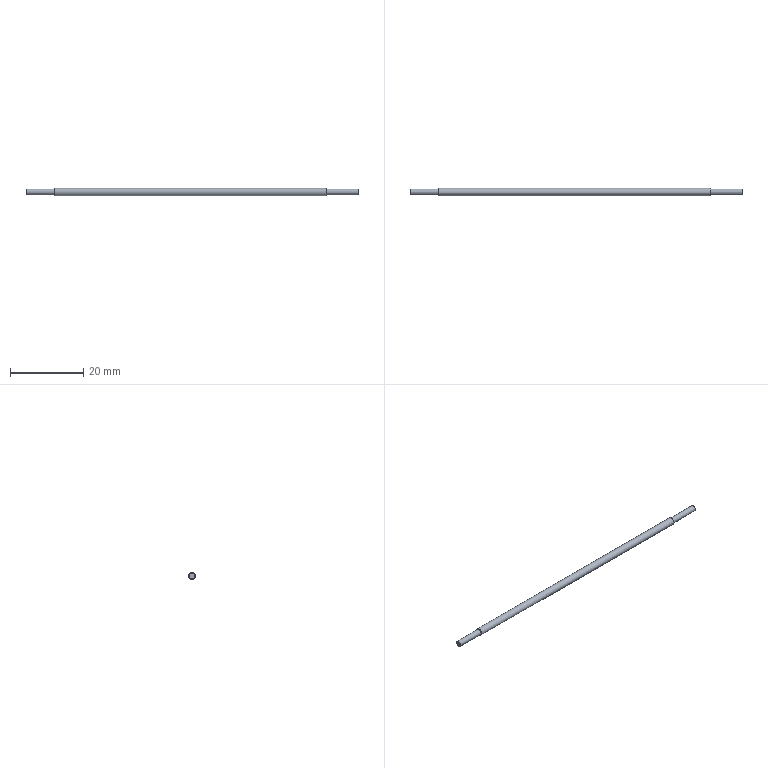Component | NX | LONG_SHAFT | 1 solid | 7 faces | box 90.9 x 2 x 2 mm | volume 267 mm3 | plane 4 | cylinder 3 | commonest cylinder face diameters 1.6 x2 2 x1
STEP:
#1=CARTESIAN_POINT('',(0.,0.,0.));
#2=DIRECTION('',(0.,0.,1.));
#3=DIRECTION('',(1.,0.,0.));
#4=AXIS2_PLACEMENT_3D('',#1,#2,#3);
#5=CARTESIAN_POINT('',(-47.4,2.21,6.167));
#6=VERTEX_POINT('',#5);
#7=CARTESIAN_POINT('',(-47.4,0.6405,6.477));
#8=VERTEX_POINT('',#7);
#9=CARTESIAN_POINT('',(-47.4,1.425,6.322));
#10=DIRECTION('',(-1.,0.,-0.));
#11=DIRECTION('',(0.,0.9811,-0.1935));
#12=AXIS2_PLACEMENT_3D('',#9,#10,#11);
#13=CIRCLE('',#12,0.8);
#14=CARTESIAN_POINT('',(-47.4,1.425,6.322));
#15=DIRECTION('',(1.,-0.,0.));
#16=DIRECTION('',(0.,0.00581,-1.));
#17=AXIS2_PLACEMENT_3D('',#14,#15,#16);
#18=PLANE('',#17);
#19=CARTESIAN_POINT('',(0.1594,0.784));
#20=CARTESIAN_POINT('',(1.517,0.508));
#21=CARTESIAN_POINT('',(0.5993,-0.53));
#22=CARTESIAN_POINT('',(-0.3187,-1.568));
#23=CARTESIAN_POINT('',(-0.7586,-0.254));
#24=CARTESIAN_POINT('',(-1.199,1.06));
#25=CARTESIAN_POINT('',(0.1594,0.784));
#26=(BOUNDED_CURVE()B_SPLINE_CURVE(2,(#19,#20,#21,#22,#23,#24,#25),.UNSPECIFIED.,.T.,.F.)B_SPLINE_CURVE_WITH_KNOTS((1,2,2,2,2,1),(-2.094,0.,2.094,4.189,6.283,8.378),.UNSPECIFIED.)CURVE()GEOMETRIC_REPRESENTATION_ITEM()RATIONAL_B_SPLINE_CURVE((1.,0.5,1.,0.5,1.,0.5,1.))REPRESENTATION_ITEM(''));
#27=(GEOMETRIC_REPRESENTATION_CONTEXT(2)PARAMETRIC_REPRESENTATION_CONTEXT()REPRESENTATION_CONTEXT('',''));
#28=DEFINITIONAL_REPRESENTATION('',(#26),#27);
#29=PCURVE('',#18,#28);
#30=CARTESIAN_POINT('',(-0.,1.425,6.322));
#31=DIRECTION('',(-1.,0.,0.));
#32=DIRECTION('',(0.,-0.9811,0.1935));
#33=AXIS2_PLACEMENT_3D('',#30,#31,#32);
#34=CYLINDRICAL_SURFACE('',#33,0.8);
#35=CARTESIAN_POINT('',(3.142,47.4));
#36=DIRECTION('',(1.,0.));
#37=VECTOR('',#36,1.);
#38=LINE('',#35,#37);
#39=(GEOMETRIC_REPRESENTATION_CONTEXT(2)PARAMETRIC_REPRESENTATION_CONTEXT()REPRESENTATION_CONTEXT('',''));
#40=DEFINITIONAL_REPRESENTATION('',(#38),#39);
#41=PCURVE('',#34,#40);
#42=SURFACE_CURVE('',#13,(#29,#41),.PCURVE_S1.);
#43=EDGE_CURVE('',#6,#8,#42,.T.);
#44=ORIENTED_EDGE('',*,*,#43,.T.);
#45=CARTESIAN_POINT('',(-47.4,1.425,6.322));
#46=DIRECTION('',(-1.,0.,-0.));
#47=DIRECTION('',(0.,0.9811,-0.1935));
#48=AXIS2_PLACEMENT_3D('',#45,#46,#47);
#49=CIRCLE('',#48,0.8);
#50=CARTESIAN_POINT('',(0.1594,0.784));
#51=CARTESIAN_POINT('',(1.517,0.508));
#52=CARTESIAN_POINT('',(0.5993,-0.53));
#53=CARTESIAN_POINT('',(-0.3187,-1.568));
#54=CARTESIAN_POINT('',(-0.7586,-0.254));
#55=CARTESIAN_POINT('',(-1.199,1.06));
#56=CARTESIAN_POINT('',(0.1594,0.784));
#57=(BOUNDED_CURVE()B_SPLINE_CURVE(2,(#50,#51,#52,#53,#54,#55,#56),.UNSPECIFIED.,.T.,.F.)B_SPLINE_CURVE_WITH_KNOTS((1,2,2,2,2,1),(-2.094,0.,2.094,4.189,6.283,8.378),.UNSPECIFIED.)CURVE()GEOMETRIC_REPRESENTATION_ITEM()RATIONAL_B_SPLINE_CURVE((1.,0.5,1.,0.5,1.,0.5,1.))REPRESENTATION_ITEM(''));
#58=(GEOMETRIC_REPRESENTATION_CONTEXT(2)PARAMETRIC_REPRESENTATION_CONTEXT()REPRESENTATION_CONTEXT('',''));
#59=DEFINITIONAL_REPRESENTATION('',(#57),#58);
#60=PCURVE('',#18,#59);
#61=CARTESIAN_POINT('',(-3.142,47.4));
#62=DIRECTION('',(1.,0.));
#63=VECTOR('',#62,1.);
#64=LINE('',#61,#63);
#65=(GEOMETRIC_REPRESENTATION_CONTEXT(2)PARAMETRIC_REPRESENTATION_CONTEXT()REPRESENTATION_CONTEXT('',''));
#66=DEFINITIONAL_REPRESENTATION('',(#64),#65);
#67=PCURVE('',#34,#66);
#68=SURFACE_CURVE('',#49,(#60,#67),.PCURVE_S1.);
#69=EDGE_CURVE('',#8,#6,#68,.T.);
#70=ORIENTED_EDGE('',*,*,#69,.T.);
#71=EDGE_LOOP('',(#44,#70));
#72=FACE_BOUND('',#71,.T.);
#73=ADVANCED_FACE('',(#72),#18,.F.);
#74=CARTESIAN_POINT('',(-39.5,0.6405,6.477));
#75=VERTEX_POINT('',#74);
#76=CARTESIAN_POINT('',(-39.5,1.425,6.322));
#77=DIRECTION('',(-1.,0.,0.));
#78=DIRECTION('',(0.,-0.9811,0.1935));
#79=AXIS2_PLACEMENT_3D('',#76,#77,#78);
#80=CIRCLE('',#79,0.8);
#81=CARTESIAN_POINT('',(0.,39.5));
#82=DIRECTION('',(1.,0.));
#83=VECTOR('',#82,1.);
#84=LINE('',#81,#83);
#85=(GEOMETRIC_REPRESENTATION_CONTEXT(2)PARAMETRIC_REPRESENTATION_CONTEXT()REPRESENTATION_CONTEXT('',''));
#86=DEFINITIONAL_REPRESENTATION('',(#84),#85);
#87=PCURVE('',#34,#86);
#88=CARTESIAN_POINT('',(-39.5,0.6405,6.477));
#89=DIRECTION('',(-1.,0.,0.));
#90=DIRECTION('',(0.,-0.9811,0.1935));
#91=AXIS2_PLACEMENT_3D('',#88,#89,#90);
#92=PLANE('',#91);
#93=CARTESIAN_POINT('',(-0.8,0.));
#94=DIRECTION('',(1.,0.));
#95=AXIS2_PLACEMENT_2D('',#93,#94);
#96=CIRCLE('',#95,0.8);
#97=(GEOMETRIC_REPRESENTATION_CONTEXT(2)PARAMETRIC_REPRESENTATION_CONTEXT()REPRESENTATION_CONTEXT('',''));
#98=DEFINITIONAL_REPRESENTATION('',(#96),#97);
#99=PCURVE('',#92,#98);
#100=SURFACE_CURVE('',#80,(#87,#99),.PCURVE_S1.);
#101=EDGE_CURVE('',#75,#75,#100,.T.);
#102=ORIENTED_EDGE('',*,*,#101,.T.);
#103=CARTESIAN_POINT('',(-39.5,0.6405,6.477));
#104=CARTESIAN_POINT('',(-47.4,0.6405,6.477));
#105=B_SPLINE_CURVE_WITH_KNOTS('',1,(#103,#104),.UNSPECIFIED.,.F.,.F.,(2,2),(39.5,47.4),.PIECEWISE_BEZIER_KNOTS.);
#106=CARTESIAN_POINT('',(6.283,0.));
#107=DIRECTION('',(0.,1.));
#108=VECTOR('',#107,1.);
#109=LINE('',#106,#108);
#110=(GEOMETRIC_REPRESENTATION_CONTEXT(2)PARAMETRIC_REPRESENTATION_CONTEXT()REPRESENTATION_CONTEXT('',''));
#111=DEFINITIONAL_REPRESENTATION('',(#109),#110);
#112=PCURVE('',#34,#111);
#113=CARTESIAN_POINT('',(0.,0.));
#114=DIRECTION('',(0.,1.));
#115=VECTOR('',#114,1.);
#116=LINE('',#113,#115);
#117=(GEOMETRIC_REPRESENTATION_CONTEXT(2)PARAMETRIC_REPRESENTATION_CONTEXT()REPRESENTATION_CONTEXT('',''));
#118=DEFINITIONAL_REPRESENTATION('',(#116),#117);
#119=PCURVE('',#34,#118);
#120=SEAM_CURVE('',#105,(#112,#119),.PCURVE_S1.);
#121=EDGE_CURVE('',#75,#8,#120,.T.);
#122=ORIENTED_EDGE('',*,*,#121,.T.);
#123=ORIENTED_EDGE('',*,*,#43,.F.);
#124=ORIENTED_EDGE('',*,*,#69,.F.);
#125=ORIENTED_EDGE('',*,*,#121,.F.);
#126=EDGE_LOOP('',(#102,#122,#123,#124,#125));
#127=FACE_BOUND('',#126,.T.);
#128=ADVANCED_FACE('',(#127),#34,.T.);
#129=CARTESIAN_POINT('',(-39.5,0.4443,6.516));
#130=VERTEX_POINT('',#129);
#131=CARTESIAN_POINT('',(-39.5,1.425,6.322));
#132=DIRECTION('',(-1.,0.,0.));
#133=DIRECTION('',(0.,-0.9811,0.1935));
#134=AXIS2_PLACEMENT_3D('',#131,#132,#133);
#135=CIRCLE('',#134,1.);
#136=CARTESIAN_POINT('',(-0.8,0.));
#137=DIRECTION('',(1.,0.));
#138=AXIS2_PLACEMENT_2D('',#136,#137);
#139=CIRCLE('',#138,1.);
#140=(GEOMETRIC_REPRESENTATION_CONTEXT(2)PARAMETRIC_REPRESENTATION_CONTEXT()REPRESENTATION_CONTEXT('',''));
#141=DEFINITIONAL_REPRESENTATION('',(#139),#140);
#142=PCURVE('',#92,#141);
#143=CARTESIAN_POINT('',(-0.,1.425,6.322));
#144=DIRECTION('',(-1.,0.,0.));
#145=DIRECTION('',(0.,-0.9811,0.1935));
#146=AXIS2_PLACEMENT_3D('',#143,#144,#145);
#147=CYLINDRICAL_SURFACE('',#146,1.);
#148=CARTESIAN_POINT('',(0.,39.5));
#149=DIRECTION('',(1.,0.));
#150=VECTOR('',#149,1.);
#151=LINE('',#148,#150);
#152=(GEOMETRIC_REPRESENTATION_CONTEXT(2)PARAMETRIC_REPRESENTATION_CONTEXT()REPRESENTATION_CONTEXT('',''));
#153=DEFINITIONAL_REPRESENTATION('',(#151),#152);
#154=PCURVE('',#147,#153);
#155=SURFACE_CURVE('',#135,(#142,#154),.PCURVE_S1.);
#156=EDGE_CURVE('',#130,#130,#155,.T.);
#157=ORIENTED_EDGE('',*,*,#156,.T.);
#158=EDGE_LOOP('',(#157));
#159=FACE_BOUND('',#158,.T.);
#160=ORIENTED_EDGE('',*,*,#101,.F.);
#161=EDGE_LOOP('',(#160));
#162=FACE_BOUND('',#161,.T.);
#163=ADVANCED_FACE('',(#159,#162),#92,.T.);
#164=CARTESIAN_POINT('',(35.,2.406,6.129));
#165=VERTEX_POINT('',#164);
#166=CARTESIAN_POINT('',(35.,0.4443,6.516));
#167=VERTEX_POINT('',#166);
#168=CARTESIAN_POINT('',(35.,1.425,6.322));
#169=DIRECTION('',(-1.,0.,0.));
#170=DIRECTION('',(0.,0.9811,-0.1935));
#171=AXIS2_PLACEMENT_3D('',#168,#169,#170);
#172=CIRCLE('',#171,1.);
#173=CARTESIAN_POINT('',(3.142,-35.));
#174=DIRECTION('',(1.,0.));
#175=VECTOR('',#174,1.);
#176=LINE('',#173,#175);
#177=(GEOMETRIC_REPRESENTATION_CONTEXT(2)PARAMETRIC_REPRESENTATION_CONTEXT()REPRESENTATION_CONTEXT('',''));
#178=DEFINITIONAL_REPRESENTATION('',(#176),#177);
#179=PCURVE('',#147,#178);
#180=CARTESIAN_POINT('',(35.,0.4443,6.516));
#181=DIRECTION('',(1.,0.,0.));
#182=DIRECTION('',(0.,0.9811,-0.1935));
#183=AXIS2_PLACEMENT_3D('',#180,#181,#182);
#184=PLANE('',#183);
#185=CARTESIAN_POINT('',(2.,0.));
#186=CARTESIAN_POINT('',(2.,-1.732));
#187=CARTESIAN_POINT('',(0.5,-0.866));
#188=CARTESIAN_POINT('',(-1.,0.));
#189=CARTESIAN_POINT('',(0.5,0.866));
#190=CARTESIAN_POINT('',(2.,1.732));
#191=CARTESIAN_POINT('',(2.,0.));
#192=(BOUNDED_CURVE()B_SPLINE_CURVE(2,(#185,#186,#187,#188,#189,#190,#191),.UNSPECIFIED.,.T.,.F.)B_SPLINE_CURVE_WITH_KNOTS((1,2,2,2,2,1),(-2.094,0.,2.094,4.189,6.283,8.378),.UNSPECIFIED.)CURVE()GEOMETRIC_REPRESENTATION_ITEM()RATIONAL_B_SPLINE_CURVE((1.,0.5,1.,0.5,1.,0.5,1.))REPRESENTATION_ITEM(''));
#193=(GEOMETRIC_REPRESENTATION_CONTEXT(2)PARAMETRIC_REPRESENTATION_CONTEXT()REPRESENTATION_CONTEXT('',''));
#194=DEFINITIONAL_REPRESENTATION('',(#192),#193);
#195=PCURVE('',#184,#194);
#196=SURFACE_CURVE('',#172,(#179,#195),.PCURVE_S1.);
#197=EDGE_CURVE('',#165,#167,#196,.T.);
#198=ORIENTED_EDGE('',*,*,#197,.T.);
#199=CARTESIAN_POINT('',(35.,0.4443,6.516));
#200=CARTESIAN_POINT('',(-39.5,0.4443,6.516));
#201=B_SPLINE_CURVE_WITH_KNOTS('',1,(#199,#200),.UNSPECIFIED.,.F.,.F.,(2,2),(-35.,39.5),.PIECEWISE_BEZIER_KNOTS.);
#202=CARTESIAN_POINT('',(6.283,0.));
#203=DIRECTION('',(0.,1.));
#204=VECTOR('',#203,1.);
#205=LINE('',#202,#204);
#206=(GEOMETRIC_REPRESENTATION_CONTEXT(2)PARAMETRIC_REPRESENTATION_CONTEXT()REPRESENTATION_CONTEXT('',''));
#207=DEFINITIONAL_REPRESENTATION('',(#205),#206);
#208=PCURVE('',#147,#207);
#209=CARTESIAN_POINT('',(0.,0.));
#210=DIRECTION('',(0.,1.));
#211=VECTOR('',#210,1.);
#212=LINE('',#209,#211);
#213=(GEOMETRIC_REPRESENTATION_CONTEXT(2)PARAMETRIC_REPRESENTATION_CONTEXT()REPRESENTATION_CONTEXT('',''));
#214=DEFINITIONAL_REPRESENTATION('',(#212),#213);
#215=PCURVE('',#147,#214);
#216=SEAM_CURVE('',#201,(#208,#215),.PCURVE_S1.);
#217=EDGE_CURVE('',#167,#130,#216,.T.);
#218=ORIENTED_EDGE('',*,*,#217,.T.);
#219=ORIENTED_EDGE('',*,*,#156,.F.);
#220=ORIENTED_EDGE('',*,*,#217,.F.);
#221=CARTESIAN_POINT('',(35.,1.425,6.322));
#222=DIRECTION('',(-1.,0.,0.));
#223=DIRECTION('',(0.,0.9811,-0.1935));
#224=AXIS2_PLACEMENT_3D('',#221,#222,#223);
#225=CIRCLE('',#224,1.);
#226=CARTESIAN_POINT('',(-3.142,-35.));
#227=DIRECTION('',(1.,0.));
#228=VECTOR('',#227,1.);
#229=LINE('',#226,#228);
#230=(GEOMETRIC_REPRESENTATION_CONTEXT(2)PARAMETRIC_REPRESENTATION_CONTEXT()REPRESENTATION_CONTEXT('',''));
#231=DEFINITIONAL_REPRESENTATION('',(#229),#230);
#232=PCURVE('',#147,#231);
#233=CARTESIAN_POINT('',(2.,0.));
#234=CARTESIAN_POINT('',(2.,-1.732));
#235=CARTESIAN_POINT('',(0.5,-0.866));
#236=CARTESIAN_POINT('',(-1.,0.));
#237=CARTESIAN_POINT('',(0.5,0.866));
#238=CARTESIAN_POINT('',(2.,1.732));
#239=CARTESIAN_POINT('',(2.,0.));
#240=(BOUNDED_CURVE()B_SPLINE_CURVE(2,(#233,#234,#235,#236,#237,#238,#239),.UNSPECIFIED.,.T.,.F.)B_SPLINE_CURVE_WITH_KNOTS((1,2,2,2,2,1),(-2.094,0.,2.094,4.189,6.283,8.378),.UNSPECIFIED.)CURVE()GEOMETRIC_REPRESENTATION_ITEM()RATIONAL_B_SPLINE_CURVE((1.,0.5,1.,0.5,1.,0.5,1.))REPRESENTATION_ITEM(''));
#241=(GEOMETRIC_REPRESENTATION_CONTEXT(2)PARAMETRIC_REPRESENTATION_CONTEXT()REPRESENTATION_CONTEXT('',''));
#242=DEFINITIONAL_REPRESENTATION('',(#240),#241);
#243=PCURVE('',#184,#242);
#244=SURFACE_CURVE('',#225,(#232,#243),.PCURVE_S1.);
#245=EDGE_CURVE('',#167,#165,#244,.T.);
#246=ORIENTED_EDGE('',*,*,#245,.T.);
#247=EDGE_LOOP('',(#198,#218,#219,#220,#246));
#248=FACE_BOUND('',#247,.T.);
#249=ADVANCED_FACE('',(#248),#147,.T.);
#250=CARTESIAN_POINT('',(35.,2.21,6.167));
#251=VERTEX_POINT('',#250);
#252=CARTESIAN_POINT('',(35.,0.6405,6.477));
#253=VERTEX_POINT('',#252);
#254=CARTESIAN_POINT('',(35.,1.425,6.322));
#255=DIRECTION('',(-1.,0.,0.));
#256=DIRECTION('',(0.,0.9811,-0.1935));
#257=AXIS2_PLACEMENT_3D('',#254,#255,#256);
#258=CIRCLE('',#257,0.8);
#259=CARTESIAN_POINT('',(1.8,0.));
#260=CARTESIAN_POINT('',(1.8,-1.386));
#261=CARTESIAN_POINT('',(0.6,-0.6928));
#262=CARTESIAN_POINT('',(-0.6,0.));
#263=CARTESIAN_POINT('',(0.6,0.6928));
#264=CARTESIAN_POINT('',(1.8,1.386));
#265=CARTESIAN_POINT('',(1.8,0.));
#266=(BOUNDED_CURVE()B_SPLINE_CURVE(2,(#259,#260,#261,#262,#263,#264,#265),.UNSPECIFIED.,.T.,.F.)B_SPLINE_CURVE_WITH_KNOTS((1,2,2,2,2,1),(-2.094,0.,2.094,4.189,6.283,8.378),.UNSPECIFIED.)CURVE()GEOMETRIC_REPRESENTATION_ITEM()RATIONAL_B_SPLINE_CURVE((1.,0.5,1.,0.5,1.,0.5,1.))REPRESENTATION_ITEM(''));
#267=(GEOMETRIC_REPRESENTATION_CONTEXT(2)PARAMETRIC_REPRESENTATION_CONTEXT()REPRESENTATION_CONTEXT('',''));
#268=DEFINITIONAL_REPRESENTATION('',(#266),#267);
#269=PCURVE('',#184,#268);
#270=CARTESIAN_POINT('',(-0.,1.425,6.322));
#271=DIRECTION('',(-1.,0.,0.));
#272=DIRECTION('',(0.,-0.9811,0.1935));
#273=AXIS2_PLACEMENT_3D('',#270,#271,#272);
#274=CYLINDRICAL_SURFACE('',#273,0.8);
#275=CARTESIAN_POINT('',(3.142,-35.));
#276=DIRECTION('',(1.,0.));
#277=VECTOR('',#276,1.);
#278=LINE('',#275,#277);
#279=(GEOMETRIC_REPRESENTATION_CONTEXT(2)PARAMETRIC_REPRESENTATION_CONTEXT()REPRESENTATION_CONTEXT('',''));
#280=DEFINITIONAL_REPRESENTATION('',(#278),#279);
#281=PCURVE('',#274,#280);
#282=SURFACE_CURVE('',#258,(#269,#281),.PCURVE_S1.);
#283=EDGE_CURVE('',#251,#253,#282,.T.);
#284=ORIENTED_EDGE('',*,*,#283,.T.);
#285=CARTESIAN_POINT('',(35.,1.425,6.322));
#286=DIRECTION('',(-1.,0.,0.));
#287=DIRECTION('',(0.,0.9811,-0.1935));
#288=AXIS2_PLACEMENT_3D('',#285,#286,#287);
#289=CIRCLE('',#288,0.8);
#290=CARTESIAN_POINT('',(1.8,0.));
#291=CARTESIAN_POINT('',(1.8,-1.386));
#292=CARTESIAN_POINT('',(0.6,-0.6928));
#293=CARTESIAN_POINT('',(-0.6,0.));
#294=CARTESIAN_POINT('',(0.6,0.6928));
#295=CARTESIAN_POINT('',(1.8,1.386));
#296=CARTESIAN_POINT('',(1.8,0.));
#297=(BOUNDED_CURVE()B_SPLINE_CURVE(2,(#290,#291,#292,#293,#294,#295,#296),.UNSPECIFIED.,.T.,.F.)B_SPLINE_CURVE_WITH_KNOTS((1,2,2,2,2,1),(-2.094,0.,2.094,4.189,6.283,8.378),.UNSPECIFIED.)CURVE()GEOMETRIC_REPRESENTATION_ITEM()RATIONAL_B_SPLINE_CURVE((1.,0.5,1.,0.5,1.,0.5,1.))REPRESENTATION_ITEM(''));
#298=(GEOMETRIC_REPRESENTATION_CONTEXT(2)PARAMETRIC_REPRESENTATION_CONTEXT()REPRESENTATION_CONTEXT('',''));
#299=DEFINITIONAL_REPRESENTATION('',(#297),#298);
#300=PCURVE('',#184,#299);
#301=CARTESIAN_POINT('',(-3.142,-35.));
#302=DIRECTION('',(1.,0.));
#303=VECTOR('',#302,1.);
#304=LINE('',#301,#303);
#305=(GEOMETRIC_REPRESENTATION_CONTEXT(2)PARAMETRIC_REPRESENTATION_CONTEXT()REPRESENTATION_CONTEXT('',''));
#306=DEFINITIONAL_REPRESENTATION('',(#304),#305);
#307=PCURVE('',#274,#306);
#308=SURFACE_CURVE('',#289,(#300,#307),.PCURVE_S1.);
#309=EDGE_CURVE('',#253,#251,#308,.T.);
#310=ORIENTED_EDGE('',*,*,#309,.T.);
#311=EDGE_LOOP('',(#284,#310));
#312=FACE_BOUND('',#311,.T.);
#313=ORIENTED_EDGE('',*,*,#197,.F.);
#314=ORIENTED_EDGE('',*,*,#245,.F.);
#315=EDGE_LOOP('',(#313,#314));
#316=FACE_BOUND('',#315,.T.);
#317=ADVANCED_FACE('',(#312,#316),#184,.T.);
#318=CARTESIAN_POINT('',(43.5,0.6405,6.477));
#319=VERTEX_POINT('',#318);
#320=CARTESIAN_POINT('',(43.5,1.425,6.322));
#321=DIRECTION('',(-1.,0.,0.));
#322=DIRECTION('',(0.,-0.9811,0.1935));
#323=AXIS2_PLACEMENT_3D('',#320,#321,#322);
#324=CIRCLE('',#323,0.8);
#325=CARTESIAN_POINT('',(0.,-43.5));
#326=DIRECTION('',(1.,0.));
#327=VECTOR('',#326,1.);
#328=LINE('',#325,#327);
#329=(GEOMETRIC_REPRESENTATION_CONTEXT(2)PARAMETRIC_REPRESENTATION_CONTEXT()REPRESENTATION_CONTEXT('',''));
#330=DEFINITIONAL_REPRESENTATION('',(#328),#329);
#331=PCURVE('',#274,#330);
#332=CARTESIAN_POINT('',(43.5,0.6405,6.477));
#333=DIRECTION('',(1.,0.,0.));
#334=DIRECTION('',(0.,0.9811,-0.1935));
#335=AXIS2_PLACEMENT_3D('',#332,#333,#334);
#336=PLANE('',#335);
#337=CARTESIAN_POINT('',(0.,-0.));
#338=CARTESIAN_POINT('',(0.,1.386));
#339=CARTESIAN_POINT('',(1.2,0.6928));
#340=CARTESIAN_POINT('',(2.4,-0.));
#341=CARTESIAN_POINT('',(1.2,-0.6928));
#342=CARTESIAN_POINT('',(0.,-1.386));
#343=CARTESIAN_POINT('',(0.,-0.));
#344=(BOUNDED_CURVE()B_SPLINE_CURVE(2,(#337,#338,#339,#340,#341,#342,#343),.UNSPECIFIED.,.T.,.F.)B_SPLINE_CURVE_WITH_KNOTS((1,2,2,2,2,1),(-2.094,0.,2.094,4.189,6.283,8.378),.UNSPECIFIED.)CURVE()GEOMETRIC_REPRESENTATION_ITEM()RATIONAL_B_SPLINE_CURVE((1.,0.5,1.,0.5,1.,0.5,1.))REPRESENTATION_ITEM(''));
#345=(GEOMETRIC_REPRESENTATION_CONTEXT(2)PARAMETRIC_REPRESENTATION_CONTEXT()REPRESENTATION_CONTEXT('',''));
#346=DEFINITIONAL_REPRESENTATION('',(#344),#345);
#347=PCURVE('',#336,#346);
#348=SURFACE_CURVE('',#324,(#331,#347),.PCURVE_S1.);
#349=EDGE_CURVE('',#319,#319,#348,.T.);
#350=ORIENTED_EDGE('',*,*,#349,.T.);
#351=CARTESIAN_POINT('',(43.5,0.6405,6.477));
#352=CARTESIAN_POINT('',(35.,0.6405,6.477));
#353=B_SPLINE_CURVE_WITH_KNOTS('',1,(#351,#352),.UNSPECIFIED.,.F.,.F.,(2,2),(-43.5,-35.),.PIECEWISE_BEZIER_KNOTS.);
#354=CARTESIAN_POINT('',(6.283,0.));
#355=DIRECTION('',(0.,1.));
#356=VECTOR('',#355,1.);
#357=LINE('',#354,#356);
#358=(GEOMETRIC_REPRESENTATION_CONTEXT(2)PARAMETRIC_REPRESENTATION_CONTEXT()REPRESENTATION_CONTEXT('',''));
#359=DEFINITIONAL_REPRESENTATION('',(#357),#358);
#360=PCURVE('',#274,#359);
#361=CARTESIAN_POINT('',(0.,0.));
#362=DIRECTION('',(0.,1.));
#363=VECTOR('',#362,1.);
#364=LINE('',#361,#363);
#365=(GEOMETRIC_REPRESENTATION_CONTEXT(2)PARAMETRIC_REPRESENTATION_CONTEXT()REPRESENTATION_CONTEXT('',''));
#366=DEFINITIONAL_REPRESENTATION('',(#364),#365);
#367=PCURVE('',#274,#366);
#368=SEAM_CURVE('',#353,(#360,#367),.PCURVE_S1.);
#369=EDGE_CURVE('',#319,#253,#368,.T.);
#370=ORIENTED_EDGE('',*,*,#369,.T.);
#371=ORIENTED_EDGE('',*,*,#283,.F.);
#372=ORIENTED_EDGE('',*,*,#309,.F.);
#373=ORIENTED_EDGE('',*,*,#369,.F.);
#374=EDGE_LOOP('',(#350,#370,#371,#372,#373));
#375=FACE_BOUND('',#374,.T.);
#376=ADVANCED_FACE('',(#375),#274,.T.);
#377=ORIENTED_EDGE('',*,*,#349,.F.);
#378=EDGE_LOOP('',(#377));
#379=FACE_BOUND('',#378,.T.);
#380=ADVANCED_FACE('',(#379),#336,.T.);
#381=CLOSED_SHELL('',(#73,#128,#163,#249,#317,#376,#380));
#382=MANIFOLD_SOLID_BREP('',#381);
#383=(LENGTH_UNIT()NAMED_UNIT(*)SI_UNIT(.MILLI.,.METRE.));
#384=UNCERTAINTY_MEASURE_WITH_UNIT(LENGTH_MEASURE(0.000005),#383,'','');
#385=(NAMED_UNIT(*)PLANE_ANGLE_UNIT()SI_UNIT($,.RADIAN.));
#386=(NAMED_UNIT(*)SI_UNIT($,.STERADIAN.)SOLID_ANGLE_UNIT());
#387=(GEOMETRIC_REPRESENTATION_CONTEXT(3)GLOBAL_UNCERTAINTY_ASSIGNED_CONTEXT((#384))GLOBAL_UNIT_ASSIGNED_CONTEXT((#383,#385,#386))REPRESENTATION_CONTEXT('',''));
#388=ADVANCED_BREP_SHAPE_REPRESENTATION('',(#4,#382),#387);